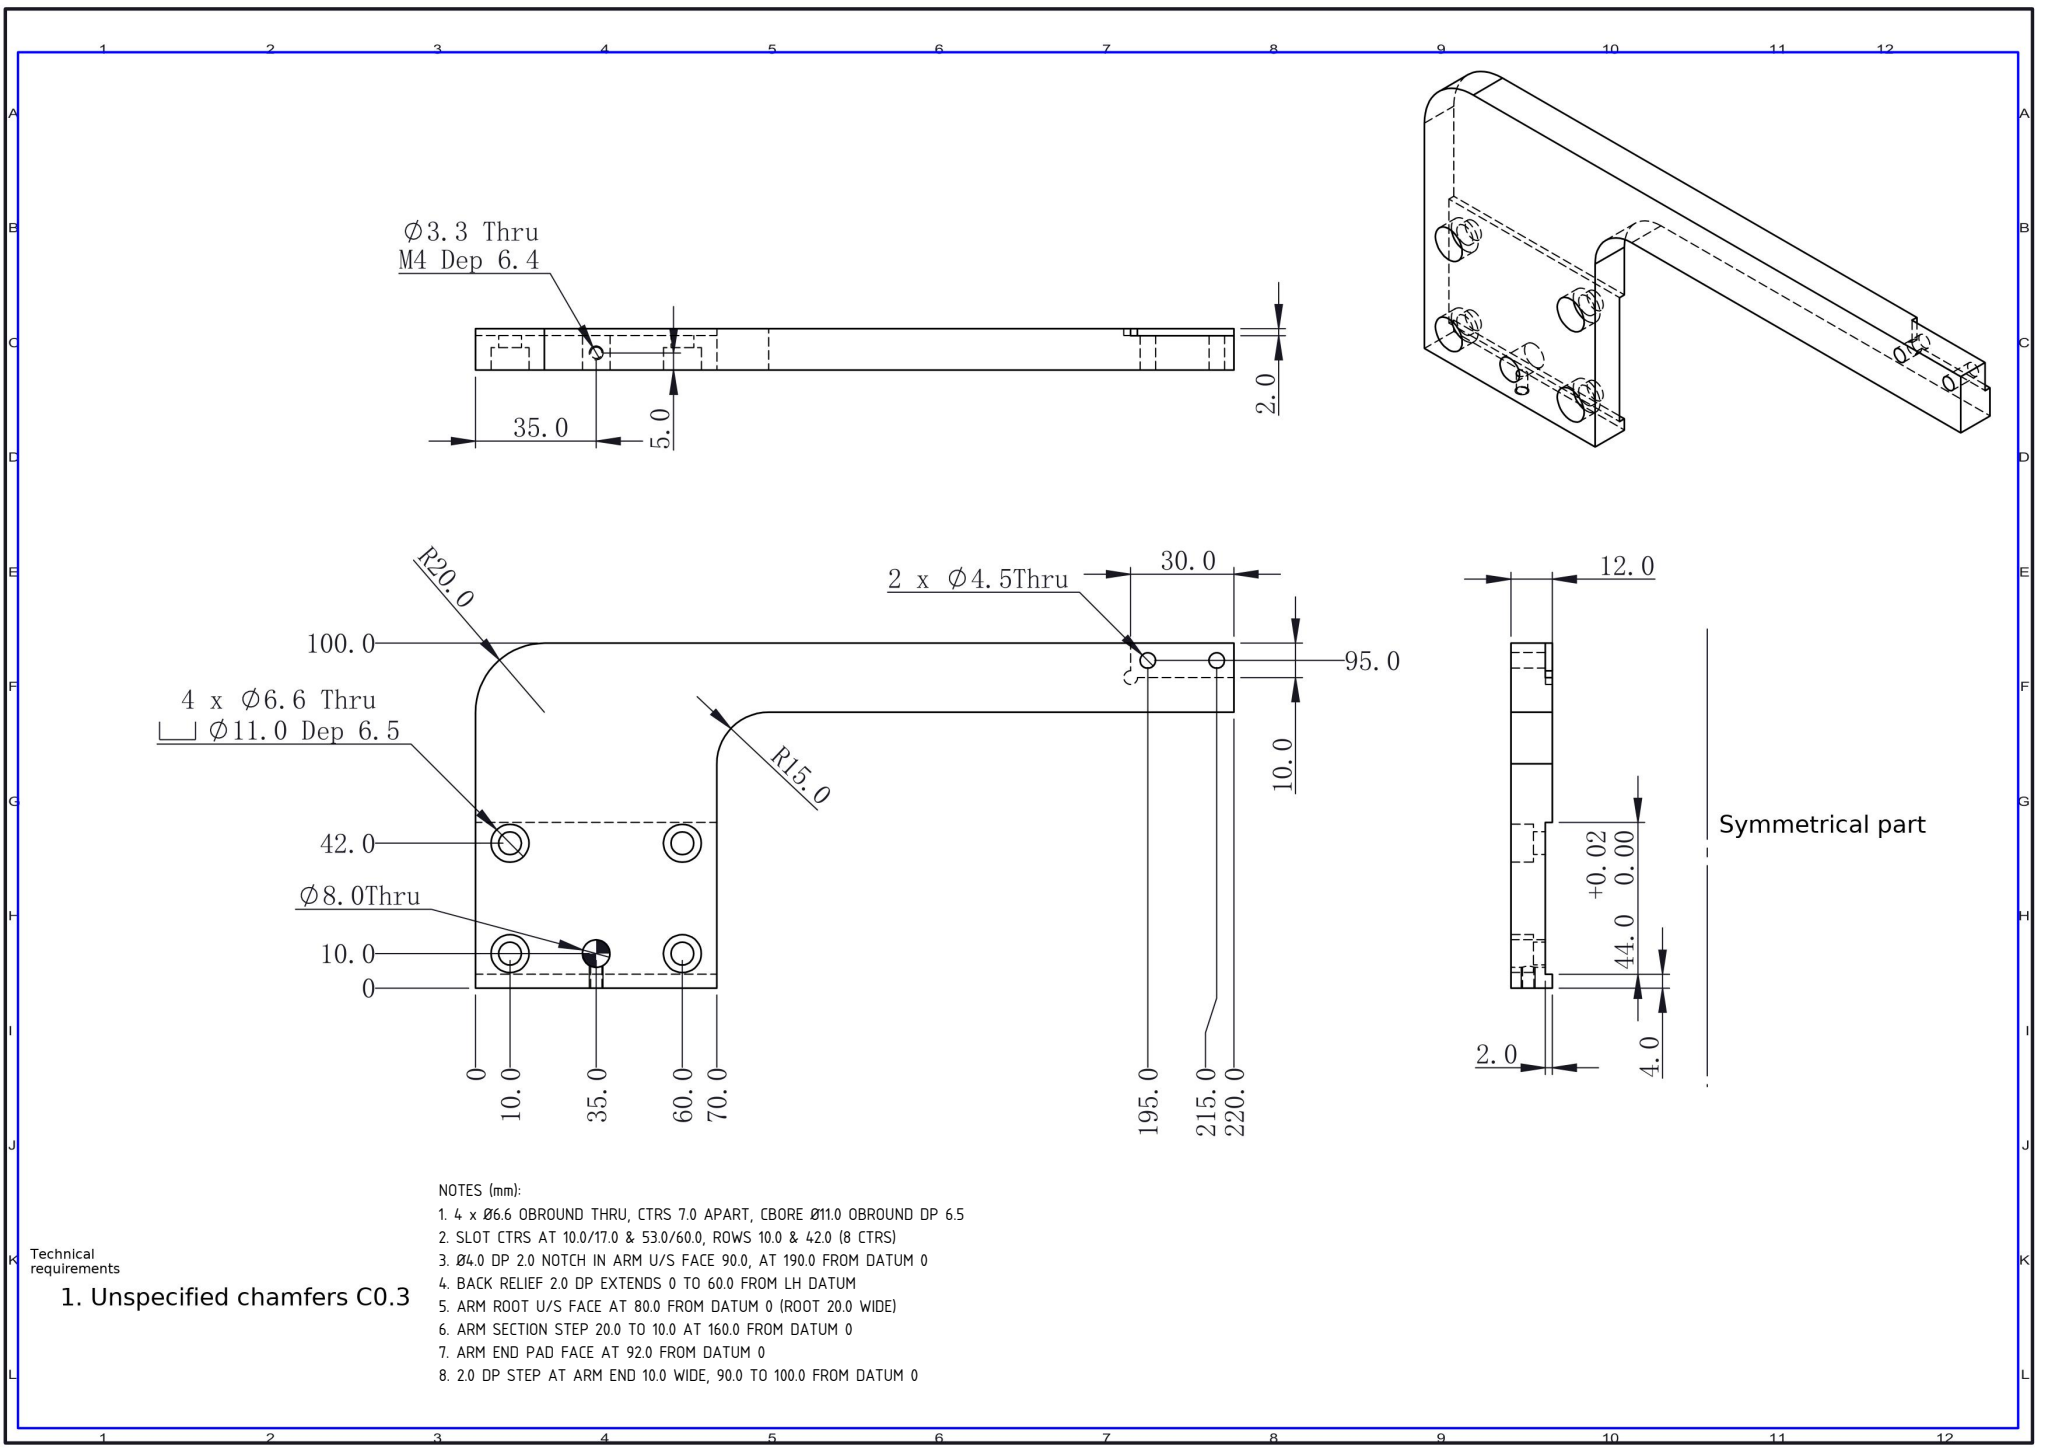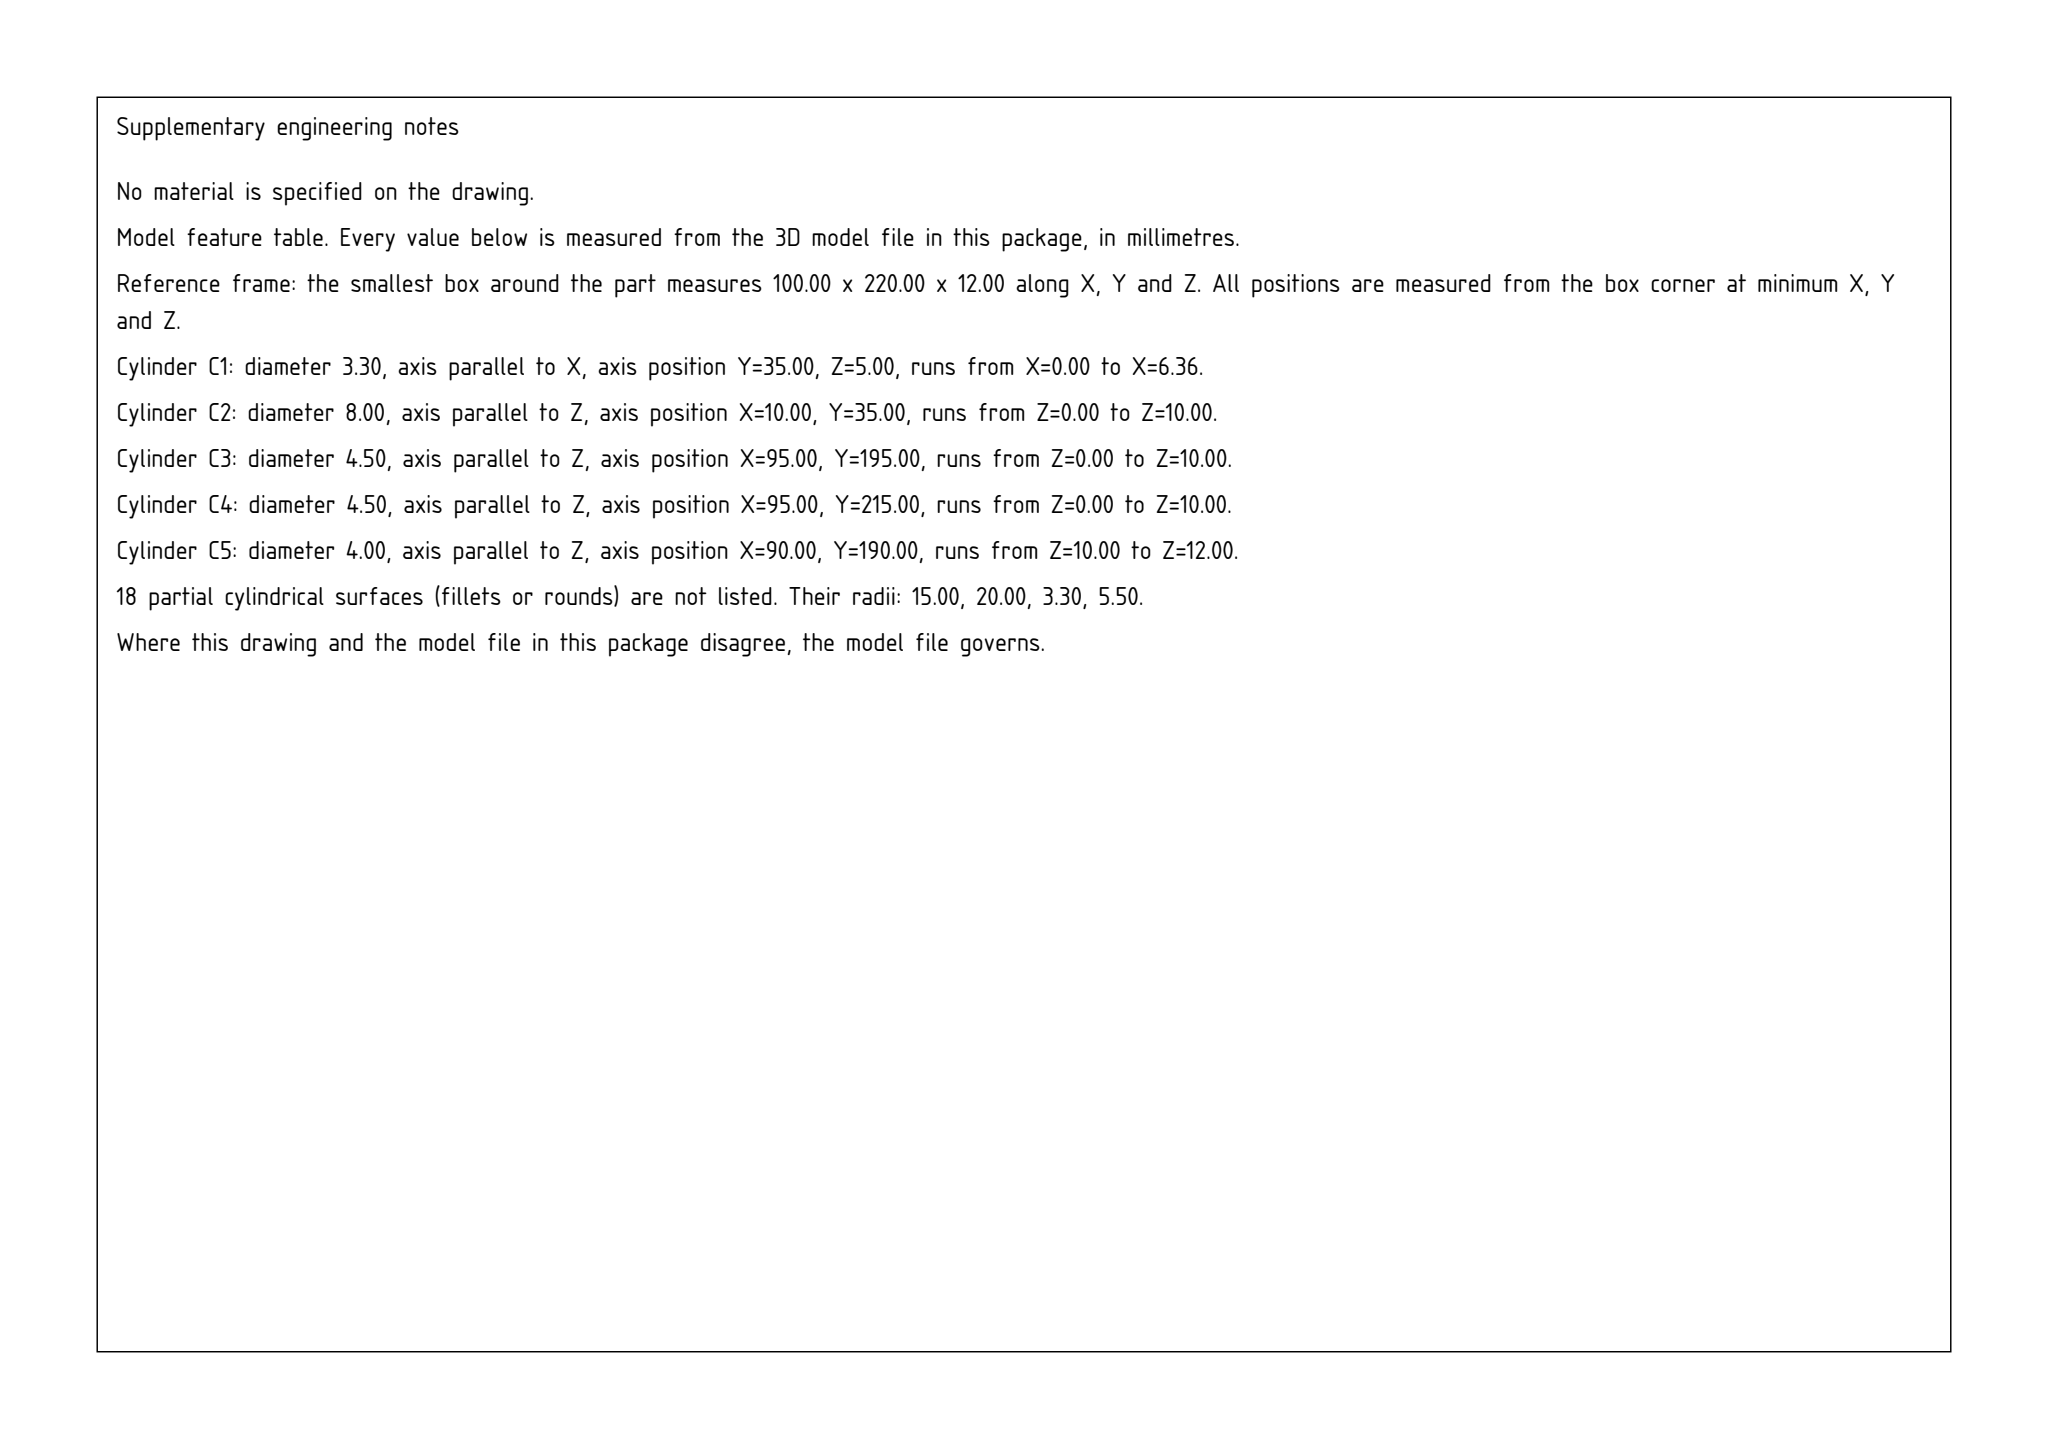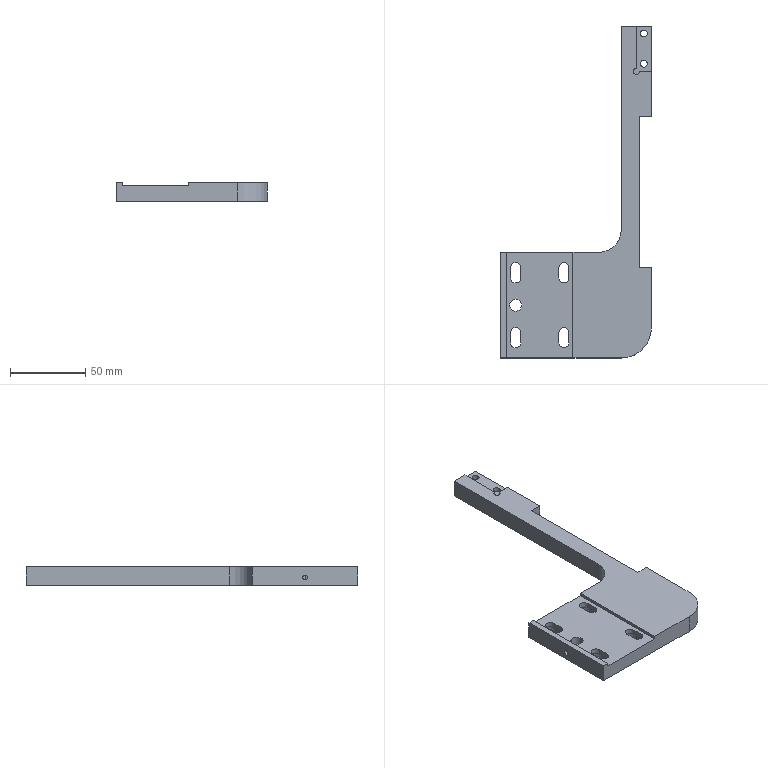Part | SolidWorks | mm | 1 solid | 82 faces | box 100 x 220 x 12 mm | volume 96699 mm3 | plane 47 | cylinder 27 | cone 8 | commonest cylinder face diameters 6.6 x8 11 x8 4.5 x4 3.3 x2 8 x2 30 x1 4 x1 40 x1
Drawing notes:
4 x Ø6.6 OBROUND THRU, CTRS 7.0 APART, CBORE Ø11.0 OBROUND DP 6.5 | from the solid: Ø6.6 pairs at y=10/17 and y=53/60 (7.0 apart) on x=10 & 42; matching Ø11 c'bores ↧6.48 (6.5)
SLOT CTRS AT 10.0/17.0 & 53.0/60.0, ROWS 10.0 & 42.0 (8 CTRS) | from the solid: 8 x Ø6.6 + 8 x Ø11 centres: (10,10)(10,17)(10,53)(10,60)(42,10)(42,17)(42,53)(42,60) = 4 slots
Ø4.0 DP 2.0 NOTCH IN ARM U/S FACE 90.0, AT 190.0 FROM DATUM 0 | from the solid: cylinder Ø4.0 axis z at (x=90, y=190), length 2.0; x-plane 90.0 = arm underside, y-plane 190.0
BACK RELIEF 2.0 DP EXTENDS 0 TO 60.0 FROM LH DATUM | from the solid: y-planes 0.0 and 60.0 bound the 2.0 deep relief (x 4.0 to 48.0 = 44.0 wide)
ARM ROOT U/S FACE AT 80.0 FROM DATUM 0 (ROOT 20.0 WIDE) | from the solid: x-plane 80.0 with outer face x=100.0 gives 20.0 root section
ARM SECTION STEP 20.0 TO 10.0 AT 160.0 FROM DATUM 0 | from the solid: y-plane 160.0 separates x=80 root face from x=90 end-section face (10.0 wide)
ARM END PAD FACE AT 92.0 FROM DATUM 0 | from the solid: x-plane 92.0 in arm end region
2.0 DP STEP AT ARM END 10.0 WIDE, 90.0 TO 100.0 FROM DATUM 0 | from the solid: z-planes 10.0 and 12.0 (2.0 deep) over y 190.0-220.0, x 90.0-100.0